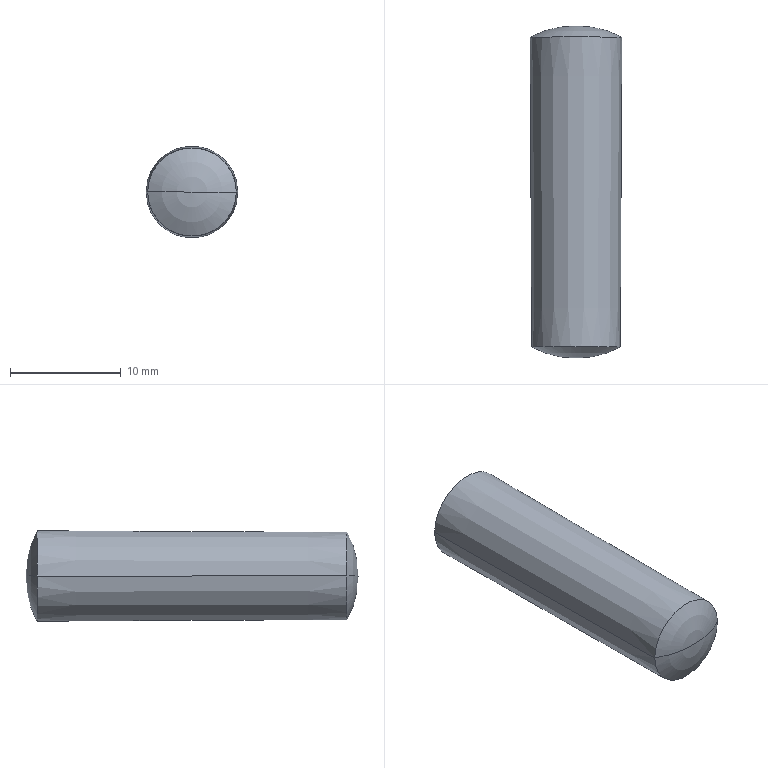Component | SolidWorks | GB_T117-2000[TaperPin8_30]-2 | 1 solid | 6 faces | box 8.28 x 30 x 8.28 mm | volume 1511 mm3 | torus 4 | cone 2
build123d program:
from build123d import *


with BuildPart() as part:
    # Sketch1 → Base-Revolve (revolve)
    with BuildSketch(Plane.XY):
        with BuildLine():
            Line((0, 0), (30, 0))
            ThreePointArc((30, 0), (29.762, -2.132), (29, -4.138))
            Line((29, -4.138), (1, -4))
            ThreePointArc((1, -4), (0.2379, -2.066), (0, 0))
        make_face()
    revolve(axis=Axis((0, 0, 0), (1, 0, 0)))


solid = part.part

# Placed as in the assembly
solid = solid.moved(Location((220, -19, 0), (0, 0, 90)))
STEP:
#1=CARTESIAN_POINT('',(8.661,0.4331,-0.));
#2=VERTEX_POINT('',#1);
#3=CARTESIAN_POINT('',(8.824,0.3937,-0.));
#4=VERTEX_POINT('',#3);
#5=CARTESIAN_POINT('',(8.666,0.09669,-0.));
#6=DIRECTION('',(0.,0.,-1.));
#7=DIRECTION('',(-1.,0.,0.));
#8=AXIS2_PLACEMENT_3D('',#5,#6,#7);
#9=CIRCLE('',#8,0.3364);
#10=EDGE_CURVE('',#2,#4,#9,.T.);
#11=ORIENTED_EDGE('',*,*,#10,.F.);
#12=CARTESIAN_POINT('',(8.498,0.3937,-0.));
#13=VERTEX_POINT('',#12);
#14=CARTESIAN_POINT('',(8.656,0.09669,-0.));
#15=DIRECTION('',(0.,0.,1.));
#16=DIRECTION('',(1.,0.,-0.));
#17=AXIS2_PLACEMENT_3D('',#14,#15,#16);
#18=CIRCLE('',#17,0.3364);
#19=EDGE_CURVE('',#2,#13,#18,.T.);
#20=ORIENTED_EDGE('',*,*,#19,.T.);
#21=CARTESIAN_POINT('',(8.661,0.3937,-0.));
#22=DIRECTION('',(0.,-1.,0.));
#23=DIRECTION('',(1.,0.,0.));
#24=AXIS2_PLACEMENT_3D('',#21,#22,#23);
#25=CIRCLE('',#24,0.1629);
#26=EDGE_CURVE('',#4,#13,#25,.T.);
#27=ORIENTED_EDGE('',*,*,#26,.F.);
#28=EDGE_LOOP('',(#11,#20,#27));
#29=FACE_OUTER_BOUND('',#28,.T.);
#30=CARTESIAN_POINT('',(8.661,0.09669,-0.));
#31=DIRECTION('',(0.,-1.,0.));
#32=DIRECTION('',(1.,0.,0.));
#33=AXIS2_PLACEMENT_3D('',#30,#31,#32);
#34=TOROIDAL_SURFACE('',#33,0.004931,0.3364);
#35=ADVANCED_FACE('',(#29),#34,.T.);
#36=CARTESIAN_POINT('',(8.819,-0.7087,-0.));
#37=VERTEX_POINT('',#36);
#38=CARTESIAN_POINT('',(8.504,-0.7087,-0.));
#39=VERTEX_POINT('',#38);
#40=CARTESIAN_POINT('',(8.661,-0.7087,-0.));
#41=DIRECTION('',(0.,-1.,0.));
#42=DIRECTION('',(1.,0.,0.));
#43=AXIS2_PLACEMENT_3D('',#40,#41,#42);
#44=CIRCLE('',#43,0.1575);
#45=EDGE_CURVE('',#37,#39,#44,.T.);
#46=ORIENTED_EDGE('',*,*,#45,.F.);
#47=CARTESIAN_POINT('',(8.819,-0.7087,-0.));
#48=DIRECTION('',(0.004936,1.,0.));
#49=VECTOR('',#48,39.37);
#50=LINE('',#47,#49);
#51=EDGE_CURVE('',#37,#4,#50,.T.);
#52=ORIENTED_EDGE('',*,*,#51,.T.);
#53=ORIENTED_EDGE('',*,*,#26,.T.);
#54=CARTESIAN_POINT('',(8.504,-0.7087,-0.));
#55=DIRECTION('',(-0.004936,1.,0.));
#56=VECTOR('',#55,39.37);
#57=LINE('',#54,#56);
#58=EDGE_CURVE('',#39,#13,#57,.T.);
#59=ORIENTED_EDGE('',*,*,#58,.F.);
#60=EDGE_LOOP('',(#46,#52,#53,#59));
#61=FACE_OUTER_BOUND('',#60,.T.);
#62=CARTESIAN_POINT('',(8.661,-0.7087,-0.));
#63=DIRECTION('',(-0.,1.,0.));
#64=DIRECTION('',(-1.,-0.,0.));
#65=AXIS2_PLACEMENT_3D('',#62,#63,#64);
#66=CONICAL_SURFACE('',#65,0.1575,0.004936);
#67=ADVANCED_FACE('',(#61),#66,.T.);
#68=ORIENTED_EDGE('',*,*,#45,.T.);
#69=CARTESIAN_POINT('',(8.661,-0.748,-0.));
#70=VERTEX_POINT('',#69);
#71=CARTESIAN_POINT('',(8.656,-0.4331,-0.));
#72=DIRECTION('',(0.,0.,1.));
#73=DIRECTION('',(1.,0.,-0.));
#74=AXIS2_PLACEMENT_3D('',#71,#72,#73);
#75=CIRCLE('',#74,0.315);
#76=EDGE_CURVE('',#39,#70,#75,.T.);
#77=ORIENTED_EDGE('',*,*,#76,.T.);
#78=CARTESIAN_POINT('',(8.666,-0.4331,-0.));
#79=DIRECTION('',(0.,0.,-1.));
#80=DIRECTION('',(-1.,0.,0.));
#81=AXIS2_PLACEMENT_3D('',#78,#79,#80);
#82=CIRCLE('',#81,0.315);
#83=EDGE_CURVE('',#37,#70,#82,.T.);
#84=ORIENTED_EDGE('',*,*,#83,.F.);
#85=EDGE_LOOP('',(#68,#77,#84));
#86=FACE_OUTER_BOUND('',#85,.T.);
#87=CARTESIAN_POINT('',(8.661,-0.4331,-0.));
#88=DIRECTION('',(0.,-1.,0.));
#89=DIRECTION('',(1.,0.,0.));
#90=AXIS2_PLACEMENT_3D('',#87,#88,#89);
#91=TOROIDAL_SURFACE('',#90,0.004931,0.315);
#92=ADVANCED_FACE('',(#86),#91,.T.);
#93=ORIENTED_EDGE('',*,*,#76,.F.);
#94=CARTESIAN_POINT('',(8.661,-0.7087,-0.));
#95=DIRECTION('',(0.,-1.,0.));
#96=DIRECTION('',(1.,0.,0.));
#97=AXIS2_PLACEMENT_3D('',#94,#95,#96);
#98=CIRCLE('',#97,0.1575);
#99=EDGE_CURVE('',#39,#37,#98,.T.);
#100=ORIENTED_EDGE('',*,*,#99,.T.);
#101=ORIENTED_EDGE('',*,*,#83,.T.);
#102=EDGE_LOOP('',(#93,#100,#101));
#103=FACE_OUTER_BOUND('',#102,.T.);
#104=CARTESIAN_POINT('',(8.661,-0.4331,-0.));
#105=DIRECTION('',(0.,-1.,0.));
#106=DIRECTION('',(1.,0.,0.));
#107=AXIS2_PLACEMENT_3D('',#104,#105,#106);
#108=TOROIDAL_SURFACE('',#107,0.004931,0.315);
#109=ADVANCED_FACE('',(#103),#108,.T.);
#110=ORIENTED_EDGE('',*,*,#51,.F.);
#111=ORIENTED_EDGE('',*,*,#99,.F.);
#112=ORIENTED_EDGE('',*,*,#58,.T.);
#113=CARTESIAN_POINT('',(8.661,0.3937,-0.));
#114=DIRECTION('',(0.,-1.,0.));
#115=DIRECTION('',(1.,0.,0.));
#116=AXIS2_PLACEMENT_3D('',#113,#114,#115);
#117=CIRCLE('',#116,0.1629);
#118=EDGE_CURVE('',#13,#4,#117,.T.);
#119=ORIENTED_EDGE('',*,*,#118,.T.);
#120=EDGE_LOOP('',(#110,#111,#112,#119));
#121=FACE_OUTER_BOUND('',#120,.T.);
#122=CARTESIAN_POINT('',(8.661,-0.7087,-0.));
#123=DIRECTION('',(-0.,1.,0.));
#124=DIRECTION('',(-1.,-0.,0.));
#125=AXIS2_PLACEMENT_3D('',#122,#123,#124);
#126=CONICAL_SURFACE('',#125,0.1575,0.004936);
#127=ADVANCED_FACE('',(#121),#126,.T.);
#128=ORIENTED_EDGE('',*,*,#19,.F.);
#129=ORIENTED_EDGE('',*,*,#10,.T.);
#130=ORIENTED_EDGE('',*,*,#118,.F.);
#131=EDGE_LOOP('',(#128,#129,#130));
#132=FACE_OUTER_BOUND('',#131,.T.);
#133=CARTESIAN_POINT('',(8.661,0.09669,-0.));
#134=DIRECTION('',(0.,-1.,0.));
#135=DIRECTION('',(1.,0.,0.));
#136=AXIS2_PLACEMENT_3D('',#133,#134,#135);
#137=TOROIDAL_SURFACE('',#136,0.004931,0.3364);
#138=ADVANCED_FACE('',(#132),#137,.T.);
#139=CLOSED_SHELL('',(#35,#67,#92,#109,#127,#138));
#140=MANIFOLD_SOLID_BREP('',#139);
#141=CARTESIAN_POINT('',(0.,0.,0.));
#142=DIRECTION('',(0.,0.,1.));
#143=DIRECTION('',(1.,0.,0.));
#144=AXIS2_PLACEMENT_3D('',#141,#142,#143);
#145=(LENGTH_UNIT()NAMED_UNIT(*)SI_UNIT($,.METRE.));
#146=LENGTH_MEASURE_WITH_UNIT(LENGTH_MEASURE(0.0254),#145);
#147=DIMENSIONAL_EXPONENTS(1.,0.,0.,0.,0.,0.,0.);
#148=(CONVERSION_BASED_UNIT('',#146)LENGTH_UNIT()NAMED_UNIT(#147));
#149=UNCERTAINTY_MEASURE_WITH_UNIT(LENGTH_MEASURE(0.00001),#148,'','');
#150=(NAMED_UNIT(*)PLANE_ANGLE_UNIT()SI_UNIT($,.RADIAN.));
#151=(NAMED_UNIT(*)SI_UNIT($,.STERADIAN.)SOLID_ANGLE_UNIT());
#152=(GEOMETRIC_REPRESENTATION_CONTEXT(3)GLOBAL_UNCERTAINTY_ASSIGNED_CONTEXT((#149))GLOBAL_UNIT_ASSIGNED_CONTEXT((#148,#150,#151))REPRESENTATION_CONTEXT('',''));
#153=ADVANCED_BREP_SHAPE_REPRESENTATION('',(#140,#144),#152);
#154=COLOUR_RGB('',0.7922,0.8196,0.9333);
#155=FILL_AREA_STYLE_COLOUR('',#154);
#156=FILL_AREA_STYLE('',(#155));
#157=SURFACE_STYLE_FILL_AREA(#156);
#158=SURFACE_SIDE_STYLE('',(#157));
#159=SURFACE_STYLE_USAGE(.BOTH.,#158);
#160=PRESENTATION_STYLE_ASSIGNMENT((#159));
#161=STYLED_ITEM('',(#160),#140);
#162=(LENGTH_UNIT()NAMED_UNIT(*)SI_UNIT($,.METRE.));
#163=LENGTH_MEASURE_WITH_UNIT(LENGTH_MEASURE(0.0254),#162);
#164=DIMENSIONAL_EXPONENTS(1.,0.,0.,0.,0.,0.,0.);
#165=(CONVERSION_BASED_UNIT('',#163)LENGTH_UNIT()NAMED_UNIT(#164));
#166=UNCERTAINTY_MEASURE_WITH_UNIT(LENGTH_MEASURE(0.00001),#165,'','');
#167=(NAMED_UNIT(*)PLANE_ANGLE_UNIT()SI_UNIT($,.RADIAN.));
#168=(NAMED_UNIT(*)SI_UNIT($,.STERADIAN.)SOLID_ANGLE_UNIT());
#169=(GEOMETRIC_REPRESENTATION_CONTEXT(3)GLOBAL_UNCERTAINTY_ASSIGNED_CONTEXT((#166))GLOBAL_UNIT_ASSIGNED_CONTEXT((#165,#167,#168))REPRESENTATION_CONTEXT('',''));
#170=MECHANICAL_DESIGN_GEOMETRIC_PRESENTATION_REPRESENTATION('',(#161),#169);
#171=PRESENTATION_LAYER_ASSIGNMENT('','',(#161));